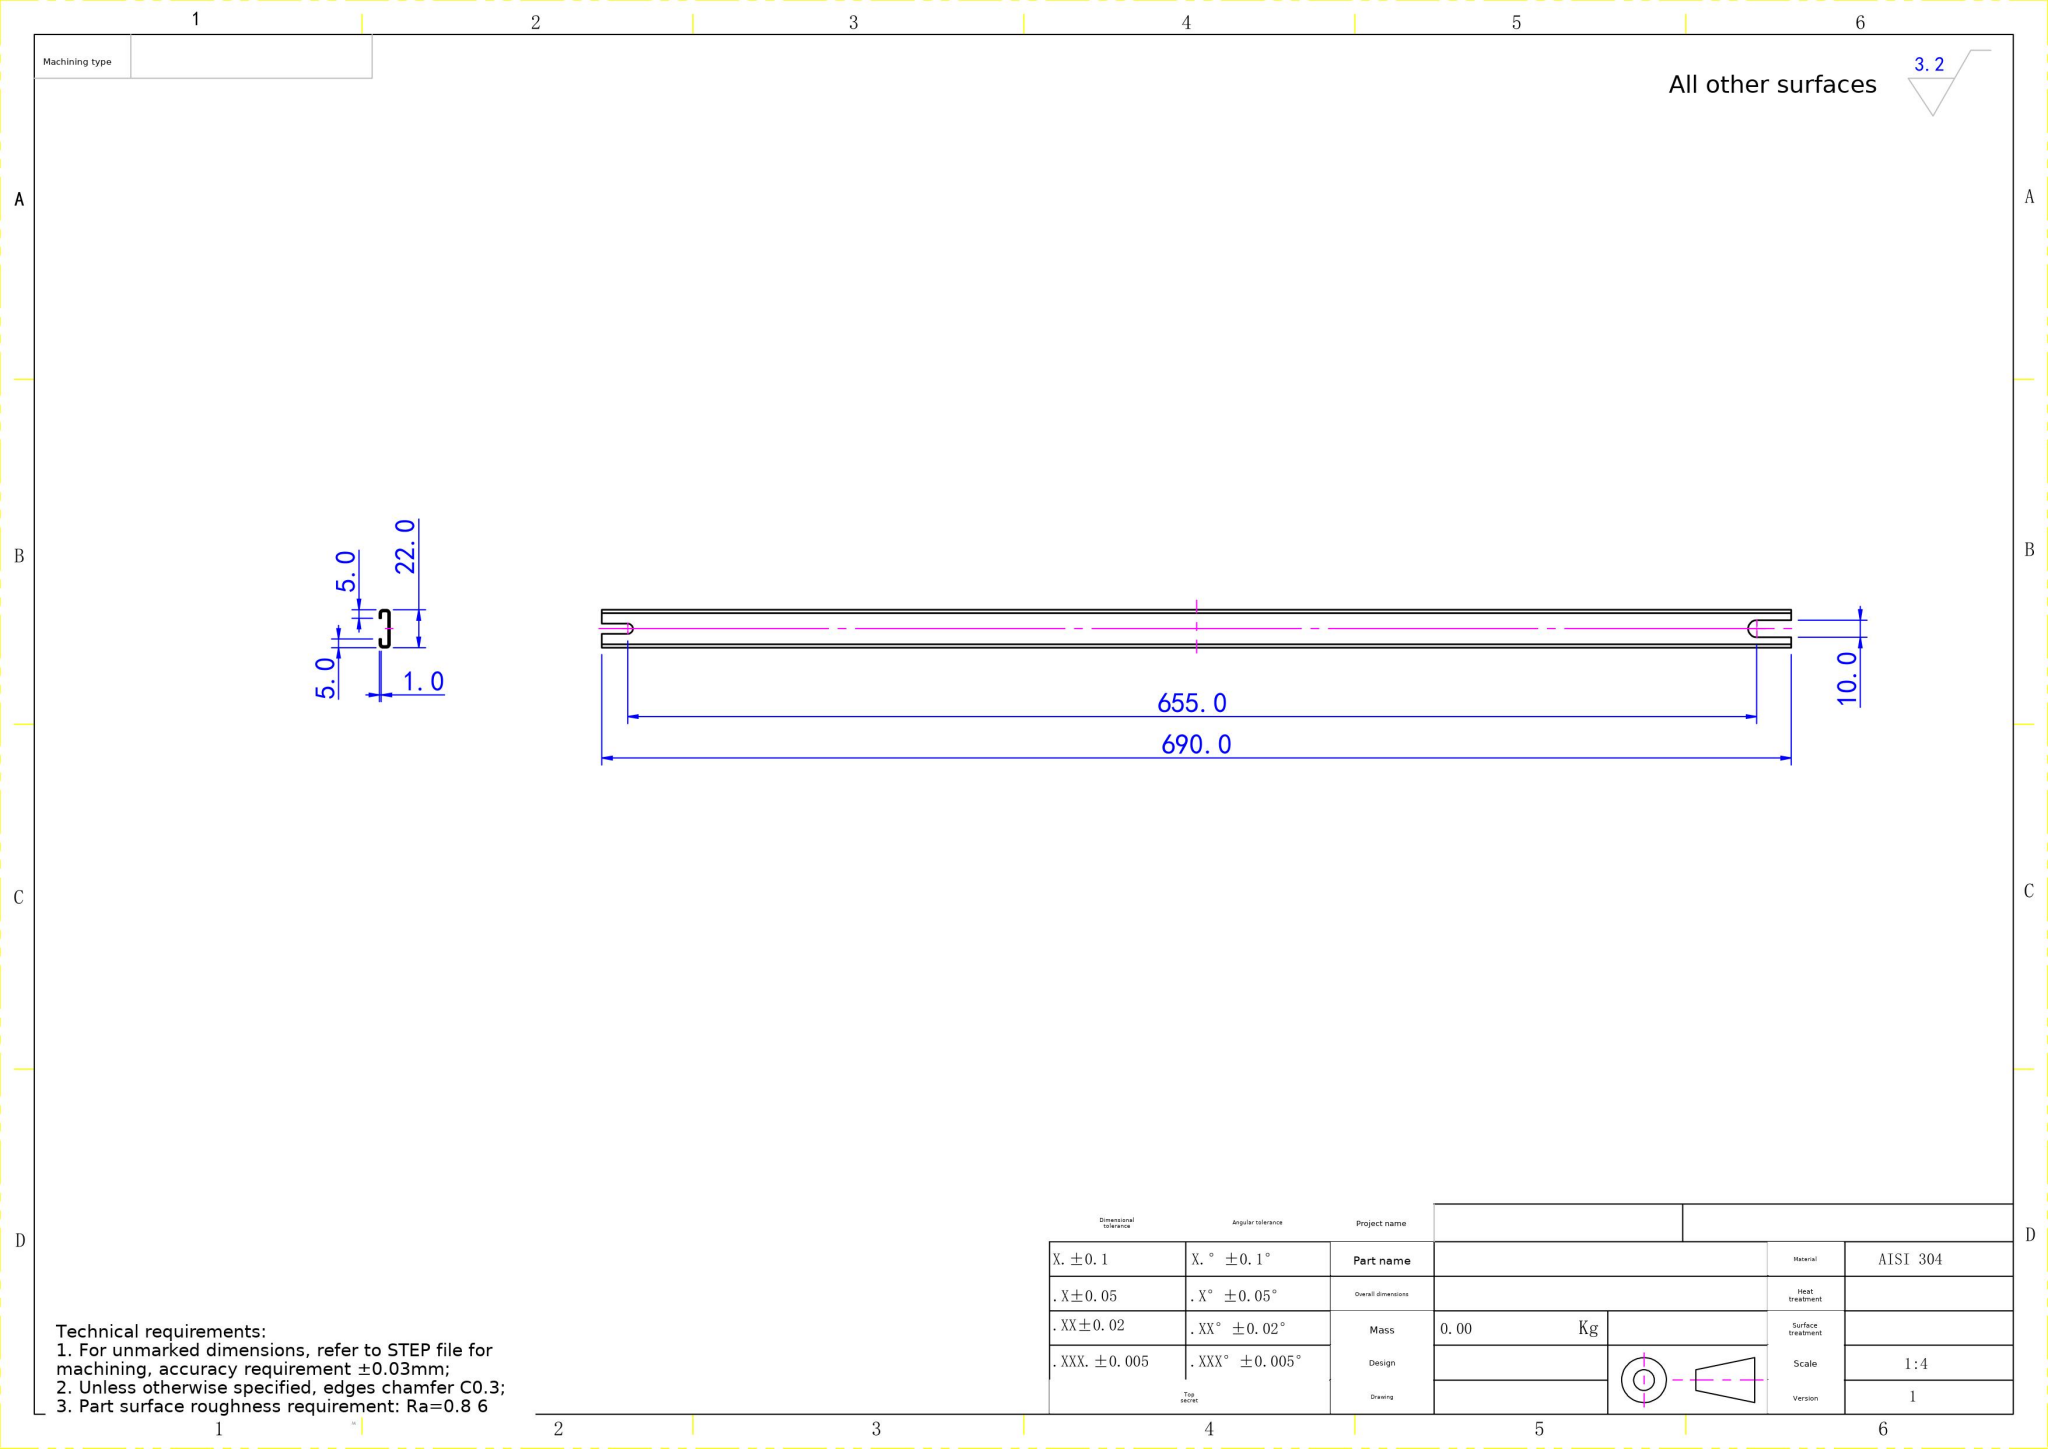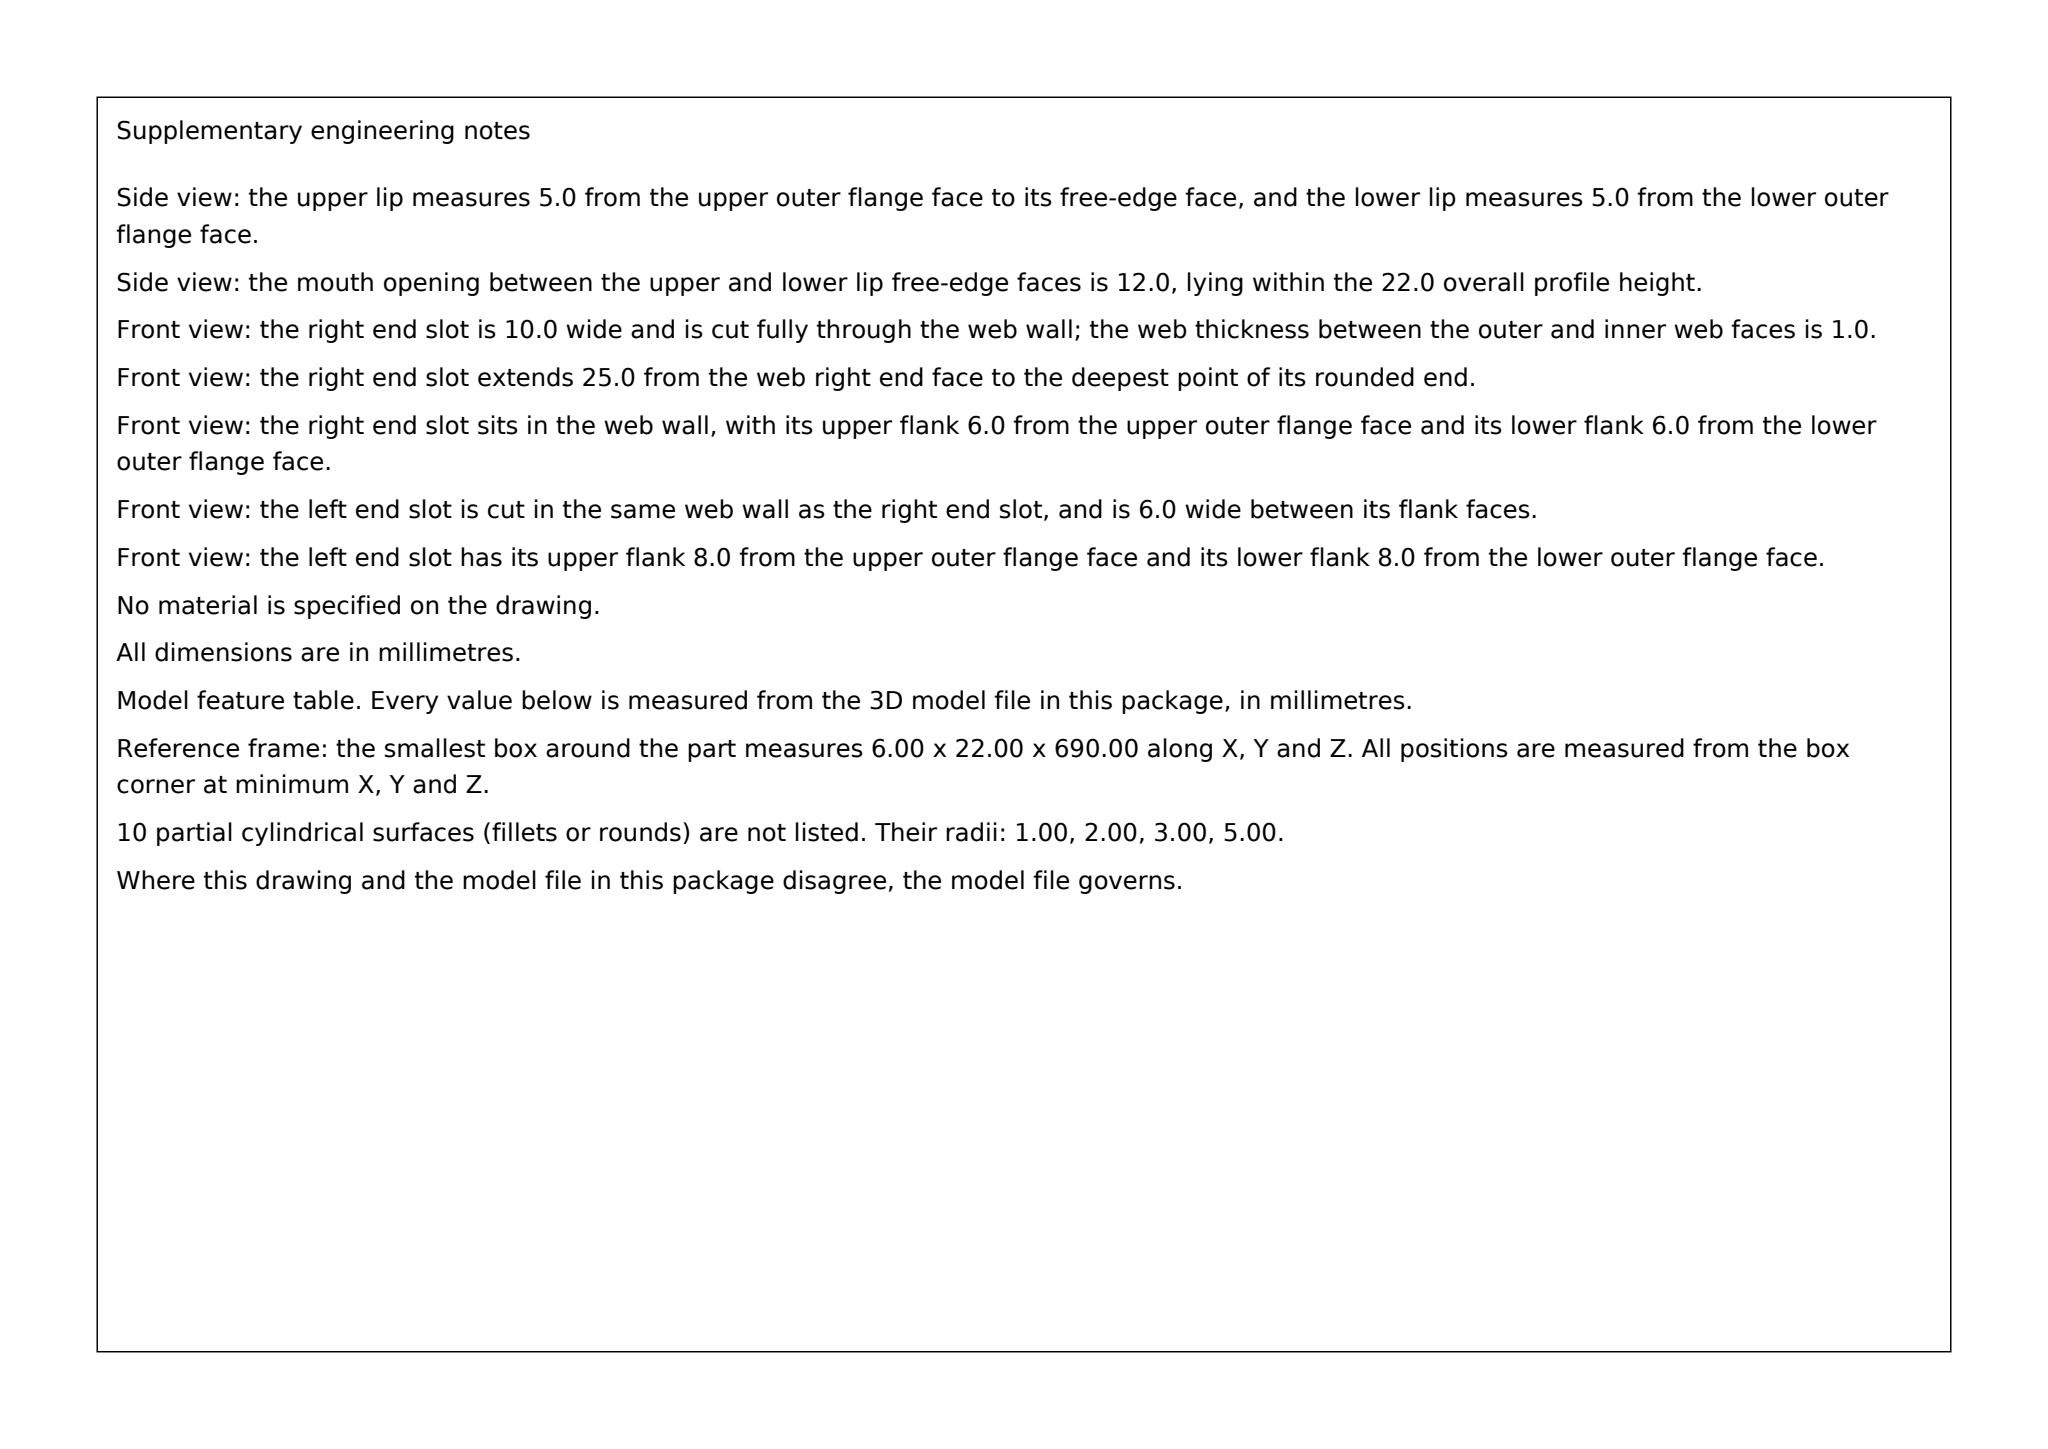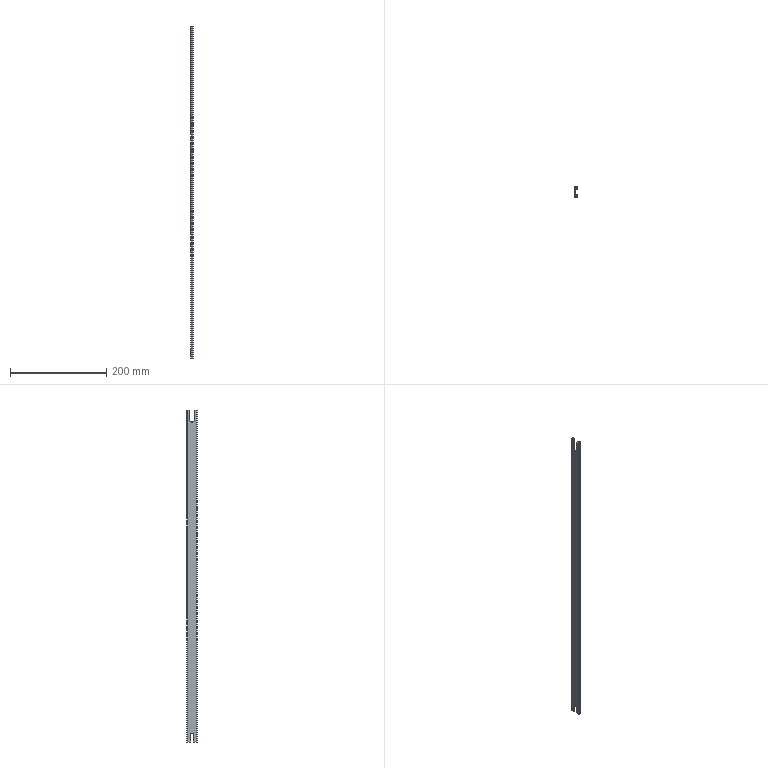Part | SolidWorks | mm | material AISI 304 | 1 solid | 47 faces | box 6 x 22 x 690 mm | volume 25480 mm3 | plane 36 | cylinder 11 | commonest cylinder face diameters 4 x4 2 x4 6 x2 10 x1
Drawing notes:
SECTION OVERALL WIDTH 6.0 (X DIR) | from the solid: bbox_xyz X = 6.0; x planes at 0.0 and 6.0
CENTRAL OPENING 6.0 BETWEEN INNER FACES | from the solid: y planes at 8.0 and 14.0 -> 6.0 gap
LH END SLOT 6.0 WIDE, THRU BOTH 1.0 WALLS | from the solid: cylinders[6.0,x,[null,11.0,15.0],1.0,count 2]
SLOT ARC CTRS: 15.0 FROM LH END, 20.0 FROM RH END | from the solid: slot z pos 15.0 and 670.0; length 690.0 -> 690-670=20.0
SECTION CORNERS: INNER R1, OUTER R2, 4 PL EA | from the solid: cyl dia 2.0 at (2,2)(2,20)(4,2)(4,20) tangent x1/y1; dia 4.0 same ctrs tangent x0/y0
SECT HT STEPS FROM BOTTOM: 1,5,6,8,14,16,17,21 OF 22.0 | from the solid: y axis_planes 0,1,5,6,8,14,16,17,21,22
RH END SLOT 10 WIDE THRU 1.0 WEB ONLY; FLANGES/LIPS INTACT | from the solid: Ø10 cyl, axis X, len 1.0 = web thk (x planes 0.0/1.0), at y=11.0, z=670
RH END SLOT OPEN TO END FACE, 20 LG TO R5 ARC CTR | from the solid: arc ctr z=670 vs bbox z=690 -> 20 from RH end; Ø10 => R5 end